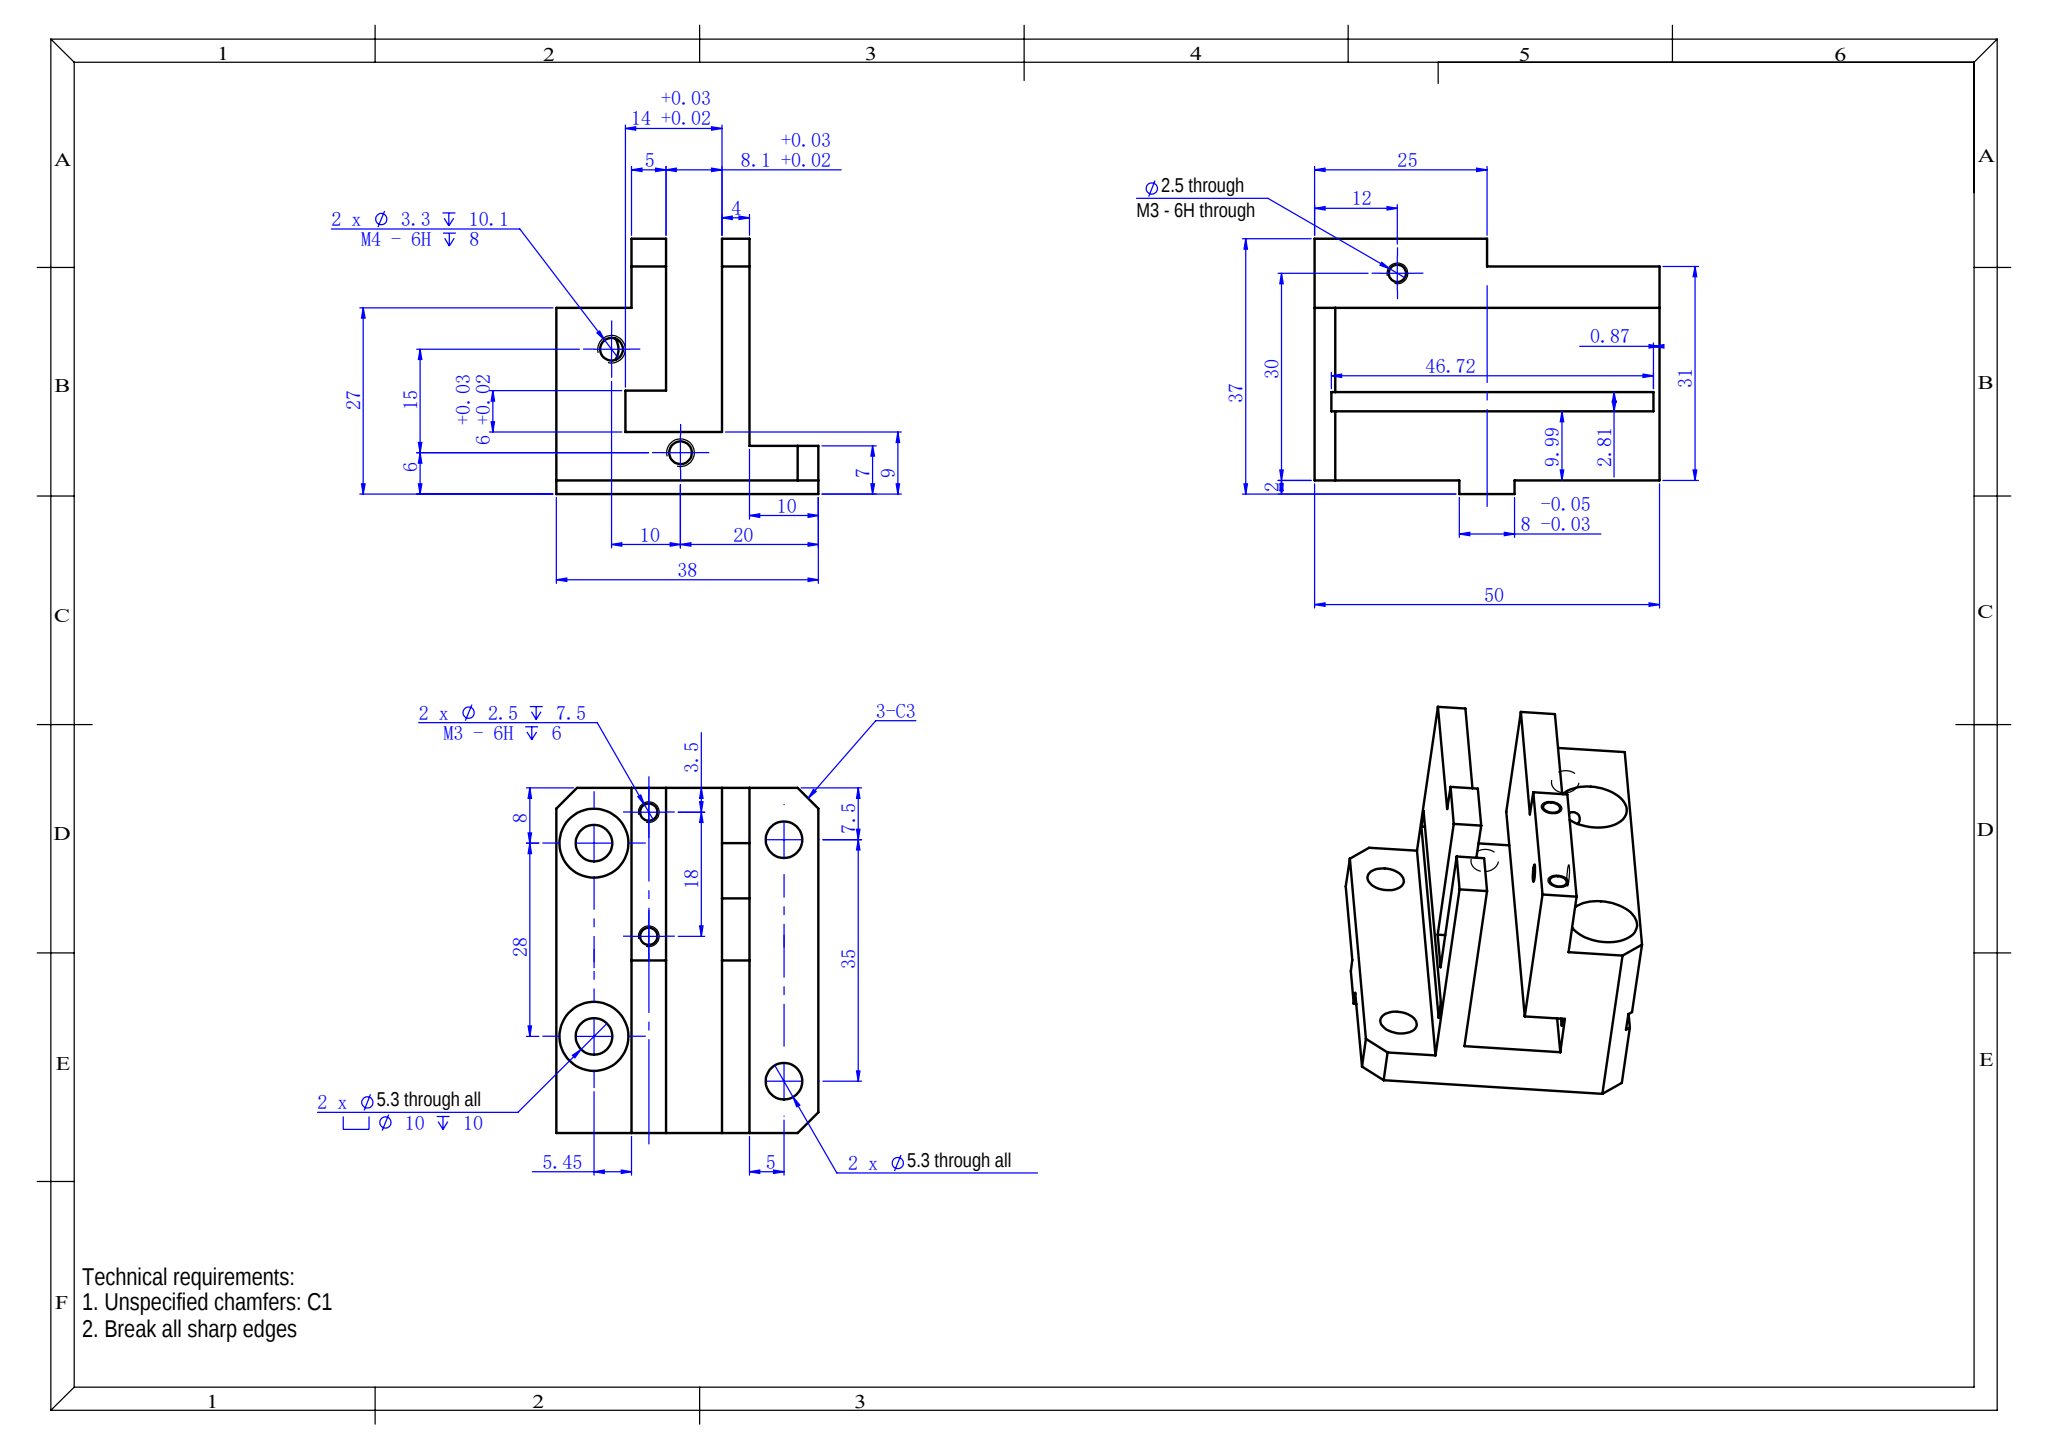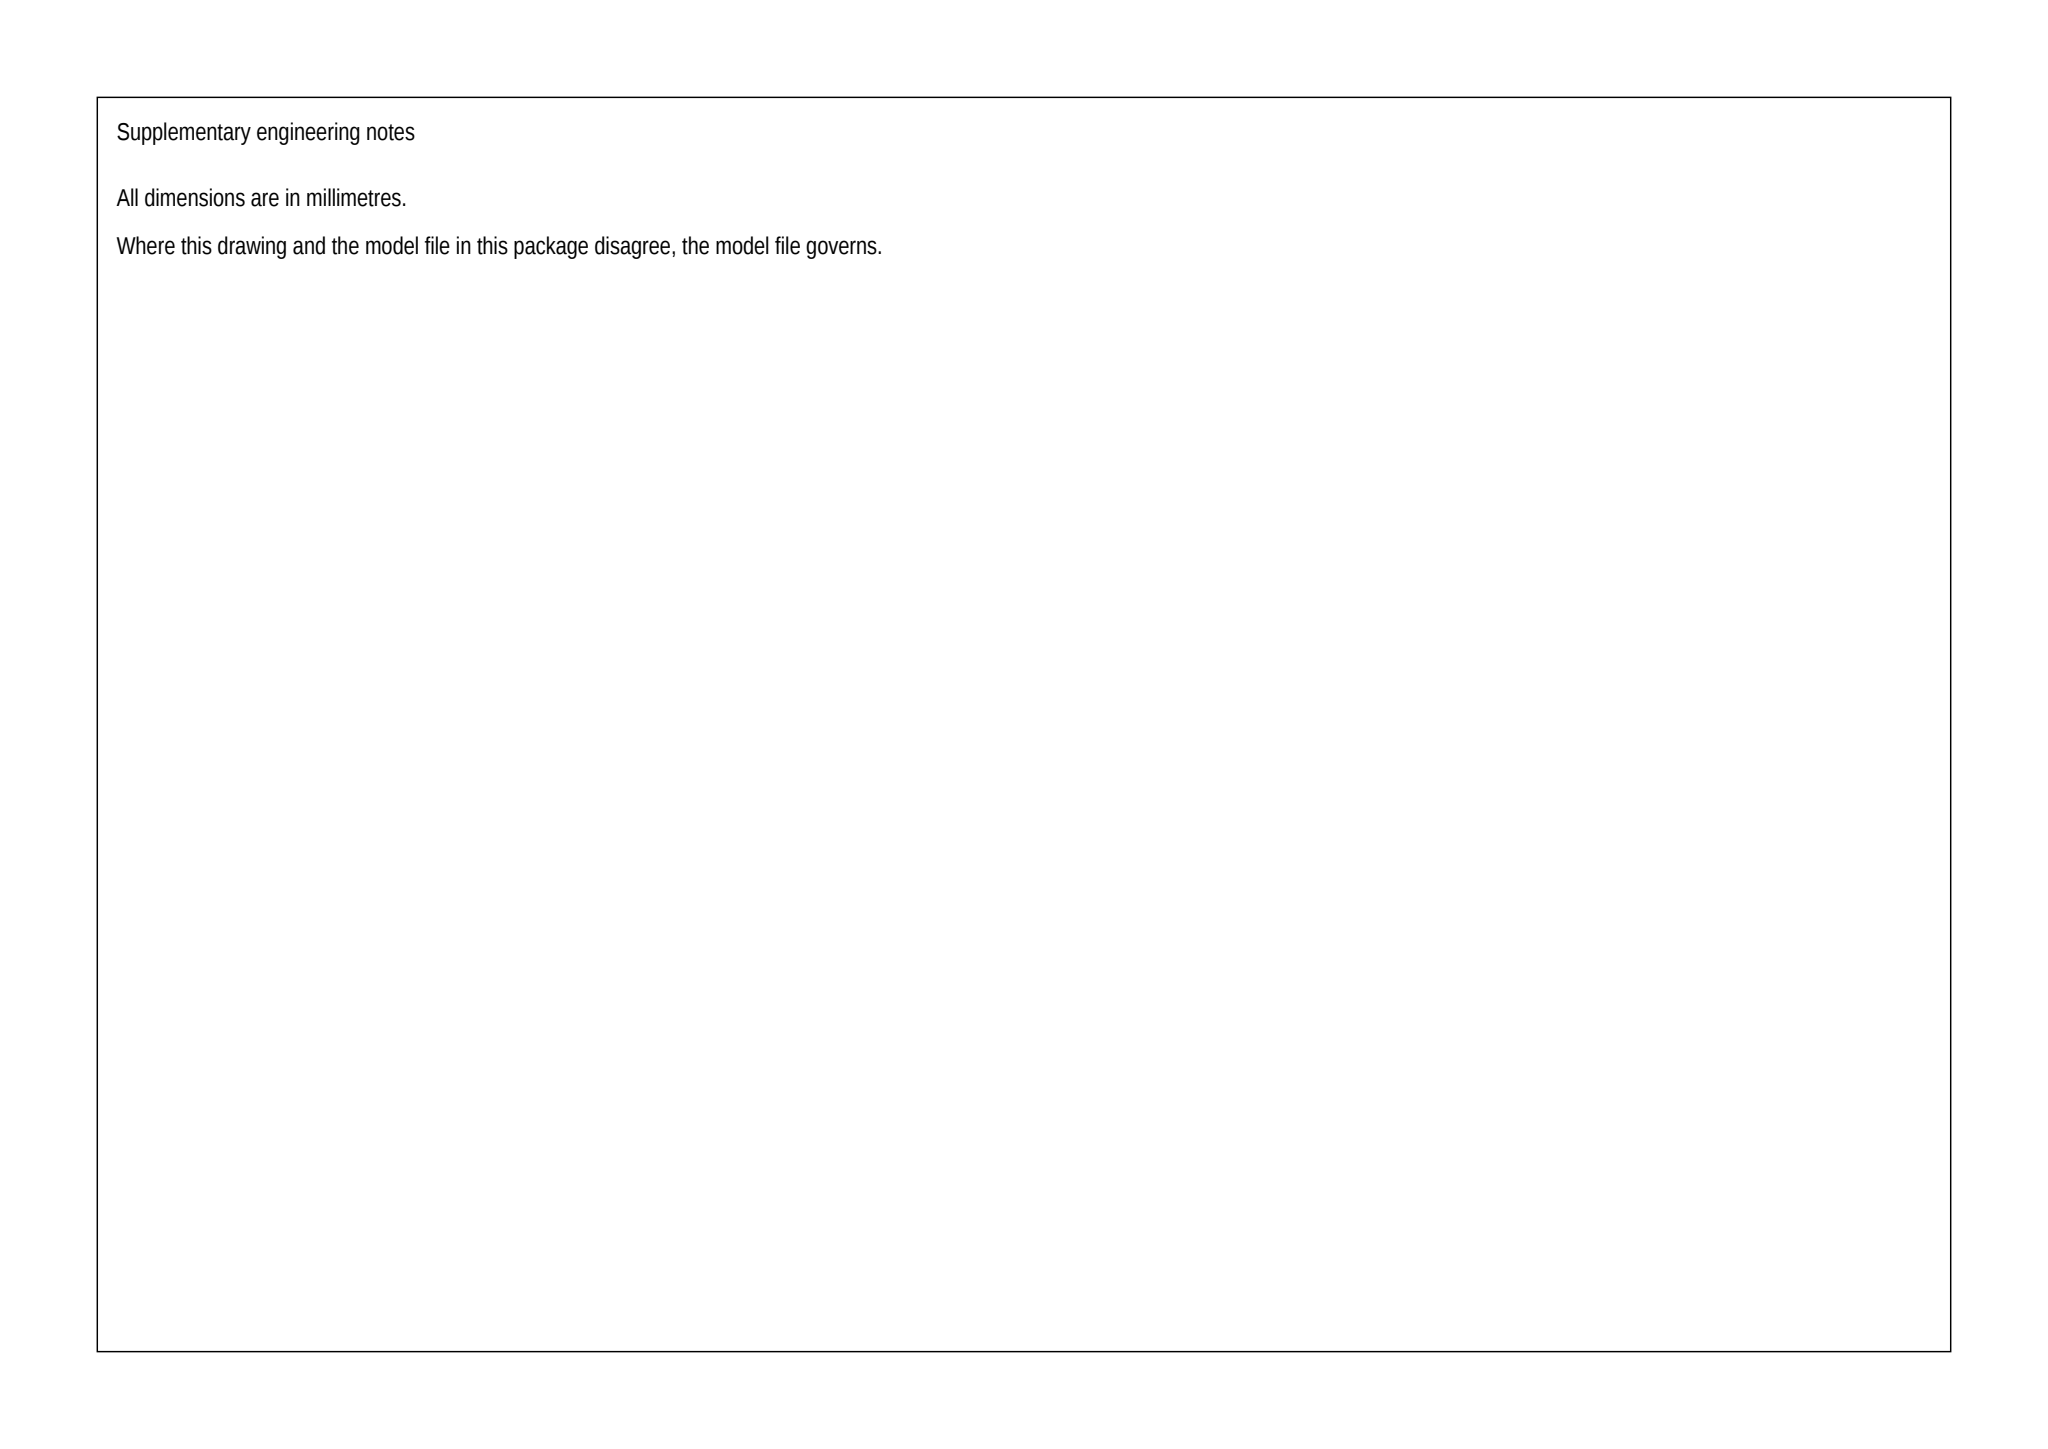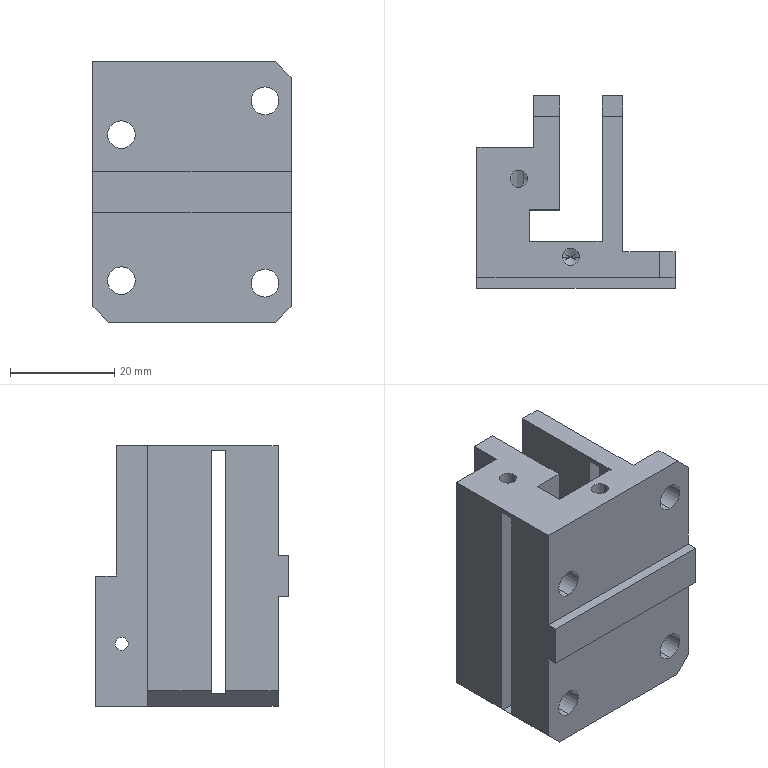Part | SolidWorks | mm | 1 solid | 75 faces | box 38 x 37 x 50 mm | volume 27411 mm3 | plane 41 | cylinder 26 | cone 8 | commonest cylinder face diameters 5.3 x12 2.5 x6 10 x4 3.3 x4
build123d program:
from build123d import *

# Parameters (mm, degrees)
SKETCH1_W                                       = 28
SKETCH1_H                                       = 35
BOSS_EXTRUDE1_DEPTH                             = 50
SKETCH2_W                                       = 8.1
SKETCH2_H                                       = 28
CUT_EXTRUDE1_DEPTH                              = 76.85
SKETCH3_W                                       = 8
SKETCH3_H                                       = 20
CUT_EXTRUDE2_DEPTH                              = 4
SKETCH4_W                                       = 6
SKETCH4_H                                       = 6
CUT_EXTRUDE3_DEPTH                              = 76.85
SKETCH5_W                                       = 25
SKETCH5_H                                       = 10
CUT_EXTRUDE4_DEPTH                              = 67.915
SKETCH8_W                                       = 10.9
SKETCH8_H                                       = 25
CUT_EXTRUDE6_DEPTH                              = 10
M4_TAPPED_HOLE1_D                               = 3.3
M4_TAPPED_HOLE1_DEPTH                           = 10.1
M4_TAPPED_HOLE1_TIP                             = 0.9914
SKETCH15_W                                      = 50
SKETCH15_H                                      = 5
BOSS_EXTRUDE2_DEPTH                             = 10
M5_HEX_SOCKET_HEAD_CAP_SCREW_CBORE1_D           = 5.3
M5_HEX_SOCKET_HEAD_CAP_SCREW_CBORE1_CBORE_D     = 10
M5_HEX_SOCKET_HEAD_CAP_SCREW_CBORE1_CBORE_DEPTH = 10
F_5_3_5_3_DIAMETER_HOLE1_D                      = 5.3
CHAMFER1_SIZE                                   = 3
M3_TAPPED_HOLE2_D                               = 2.5
M3_TAPPED_HOLE2_DEPTH                           = 7.5
M3_TAPPED_HOLE2_TIP                             = 0.7511
M3_TAPPED_HOLE3_D                               = 2.5
SKETCH27_W                                      = 5
SKETCH27_H                                      = 25
SKETCH27_W_2                                    = 4
BOSS_EXTRUDE3_DEPTH                             = 6
SKETCH28_W                                      = 8
SKETCH28_H                                      = 2
BOSS_EXTRUDE4_DEPTH                             = 38
SKETCH29_W                                      = 46.725
SKETCH29_H                                      = 2.809
CUT_EXTRUDE7_DEPTH                              = 111


with BuildPart() as part:
    # Sketch1 → Boss-Extrude1 (new body)
    with BuildSketch(Plane.XY):
        with Locations((31.384, 17.049)):
            Rectangle(SKETCH1_W, SKETCH1_H)
    extrude(amount=BOSS_EXTRUDE1_DEPTH)

    # Sketch2 → Cut-Extrude1 (cut, through all)
    with BuildSketch(Plane(origin=(0, 0, 0), x_dir=(-1, 0, 0), z_dir=(0, 0, -1))):
        with Locations((-37.334, 20.549)):
            Rectangle(SKETCH2_W, SKETCH2_H)
    extrude(amount=-CUT_EXTRUDE1_DEPTH, mode=Mode.SUBTRACT)

    # Sketch3 → Cut-Extrude2 (cut)
    with BuildSketch(Plane(origin=(45.384, 0, 0), x_dir=(0, 0, -1), z_dir=(1, 0, 0))):
        with Locations((-12, 24.549)):
            Rectangle(SKETCH3_W, SKETCH3_H)
    extrude(amount=-CUT_EXTRUDE2_DEPTH, mode=Mode.SUBTRACT)

    # Sketch4 → Cut-Extrude3 (cut, through all)
    with BuildSketch(Plane(origin=(0, 0, 0), x_dir=(-1, 0, 0), z_dir=(0, 0, -1))):
        with Locations((-30.384, 9.549)):
            Rectangle(SKETCH4_W, SKETCH4_H)
    extrude(amount=-CUT_EXTRUDE3_DEPTH, mode=Mode.SUBTRACT)

    # Sketch5 → Cut-Extrude4 (cut, through all)
    with BuildSketch(Plane(origin=(45.384, 0, 0), x_dir=(0, 0, -1), z_dir=(1, 0, 0))):
        with Locations((-37.5, 29.549)):
            Rectangle(SKETCH5_W, SKETCH5_H)
    extrude(amount=-CUT_EXTRUDE4_DEPTH, mode=Mode.SUBTRACT)

    # Sketch8 → Cut-Extrude6 (cut)
    with BuildSketch(Plane(origin=(0, 34.549, 0), x_dir=(1, 0, 0), z_dir=(0, 1, 0))):
        with Locations((22.834, -12.5)):
            Rectangle(SKETCH8_W, SKETCH8_H)
    extrude(amount=-CUT_EXTRUDE6_DEPTH, mode=Mode.SUBTRACT)

    # M4 Tapped Hole1
    with Locations(Plane.XY.offset(50)):
        with Locations((25.384, 18.549), (35.384, 3.549)):
            Hole(M4_TAPPED_HOLE1_D / 2, depth=M4_TAPPED_HOLE1_DEPTH)
            with Locations((0, 0, -(M4_TAPPED_HOLE1_DEPTH + M4_TAPPED_HOLE1_TIP / 2))):  # 118° drill point
                Cone(0, M4_TAPPED_HOLE1_D / 2, M4_TAPPED_HOLE1_TIP, mode=Mode.SUBTRACT)

    # Sketch15 → Boss-Extrude2 (add)
    with BuildSketch(Plane(origin=(45.384, 0, 0), x_dir=(0, 0, -1), z_dir=(1, 0, 0))):
        with Locations((-25, 2.049)):
            Rectangle(SKETCH15_W, SKETCH15_H)
    extrude(amount=BOSS_EXTRUDE2_DEPTH)

    # M5 Hex Socket Head Cap Screw CBORE1 (through all)
    with Locations(Plane(origin=(0, 24.549, 0), x_dir=(1, 0, 0), z_dir=(0, 1, 0))):
        with Locations((22.834, -36), (22.834, -8)):
            CounterBoreHole(M5_HEX_SOCKET_HEAD_CAP_SCREW_CBORE1_D / 2, M5_HEX_SOCKET_HEAD_CAP_SCREW_CBORE1_CBORE_D / 2, M5_HEX_SOCKET_HEAD_CAP_SCREW_CBORE1_CBORE_DEPTH)

    # 5.3 _5.3_ Diameter Hole1 (through all)
    with Locations(Plane(origin=(0, 4.549, 0), x_dir=(1, 0, 0), z_dir=(0, 1, 0))):
        with Locations((50.384, -7.5), (50.384, -42.5)):
            Hole(F_5_3_5_3_DIAMETER_HOLE1_D / 2)

    # Chamfer1
    chamfer1_edges = [part.edges().sort_by_distance(p)[0] for p in [
        (55.384, 2.049, 50),
        (55.384, 2.049, 0),
        (17.384, 12.049, 0),
    ]]
    chamfer(chamfer1_edges, length=CHAMFER1_SIZE)

    # M3 Tapped Hole2
    with Locations(Plane(origin=(0, 34.549, 0), x_dir=(1, 0, 0), z_dir=(0, 1, 0))):
        with Locations((30.784, -21.5), (30.784, -3.5)):
            Hole(M3_TAPPED_HOLE2_D / 2, depth=M3_TAPPED_HOLE2_DEPTH)
            with Locations((0, 0, -(M3_TAPPED_HOLE2_DEPTH + M3_TAPPED_HOLE2_TIP / 2))):  # 118° drill point
                Cone(0, M3_TAPPED_HOLE2_D / 2, M3_TAPPED_HOLE2_TIP, mode=Mode.SUBTRACT)

    # M3 Tapped Hole3 (through all)
    with Locations(Plane.ZY.offset(-28.284)):
        with Locations((12, 29.549)):
            Hole(M3_TAPPED_HOLE3_D / 2)

    # Sketch27 → Boss-Extrude3 (add)
    with BuildSketch(Plane(origin=(0, 24.549, 0), x_dir=(1, 0, 0), z_dir=(0, 1, 0))):
        with Locations((30.784, -37.5)):
            Rectangle(SKETCH27_W, SKETCH27_H)
        with Locations((43.384, -37.5)):
            Rectangle(SKETCH27_W_2, SKETCH27_H)
    extrude(amount=BOSS_EXTRUDE3_DEPTH)

    # Sketch28 → Boss-Extrude4 (add, through all)
    with BuildSketch(Plane.ZY.offset(-17.384)):
        with Locations((25, -1.451)):
            Rectangle(SKETCH28_W, SKETCH28_H)
    extrude(amount=-BOSS_EXTRUDE4_DEPTH)

    # Sketch29 → Cut-Extrude7 (cut)
    with BuildSketch(Plane(origin=(45.384, 0, 0), x_dir=(0, 0, -1), z_dir=(1, 0, 0))):
        with Locations((-25.771, 10.945)):
            Rectangle(SKETCH29_W, SKETCH29_H)
    extrude(amount=-CUT_EXTRUDE7_DEPTH, mode=Mode.SUBTRACT)


solid = part.part